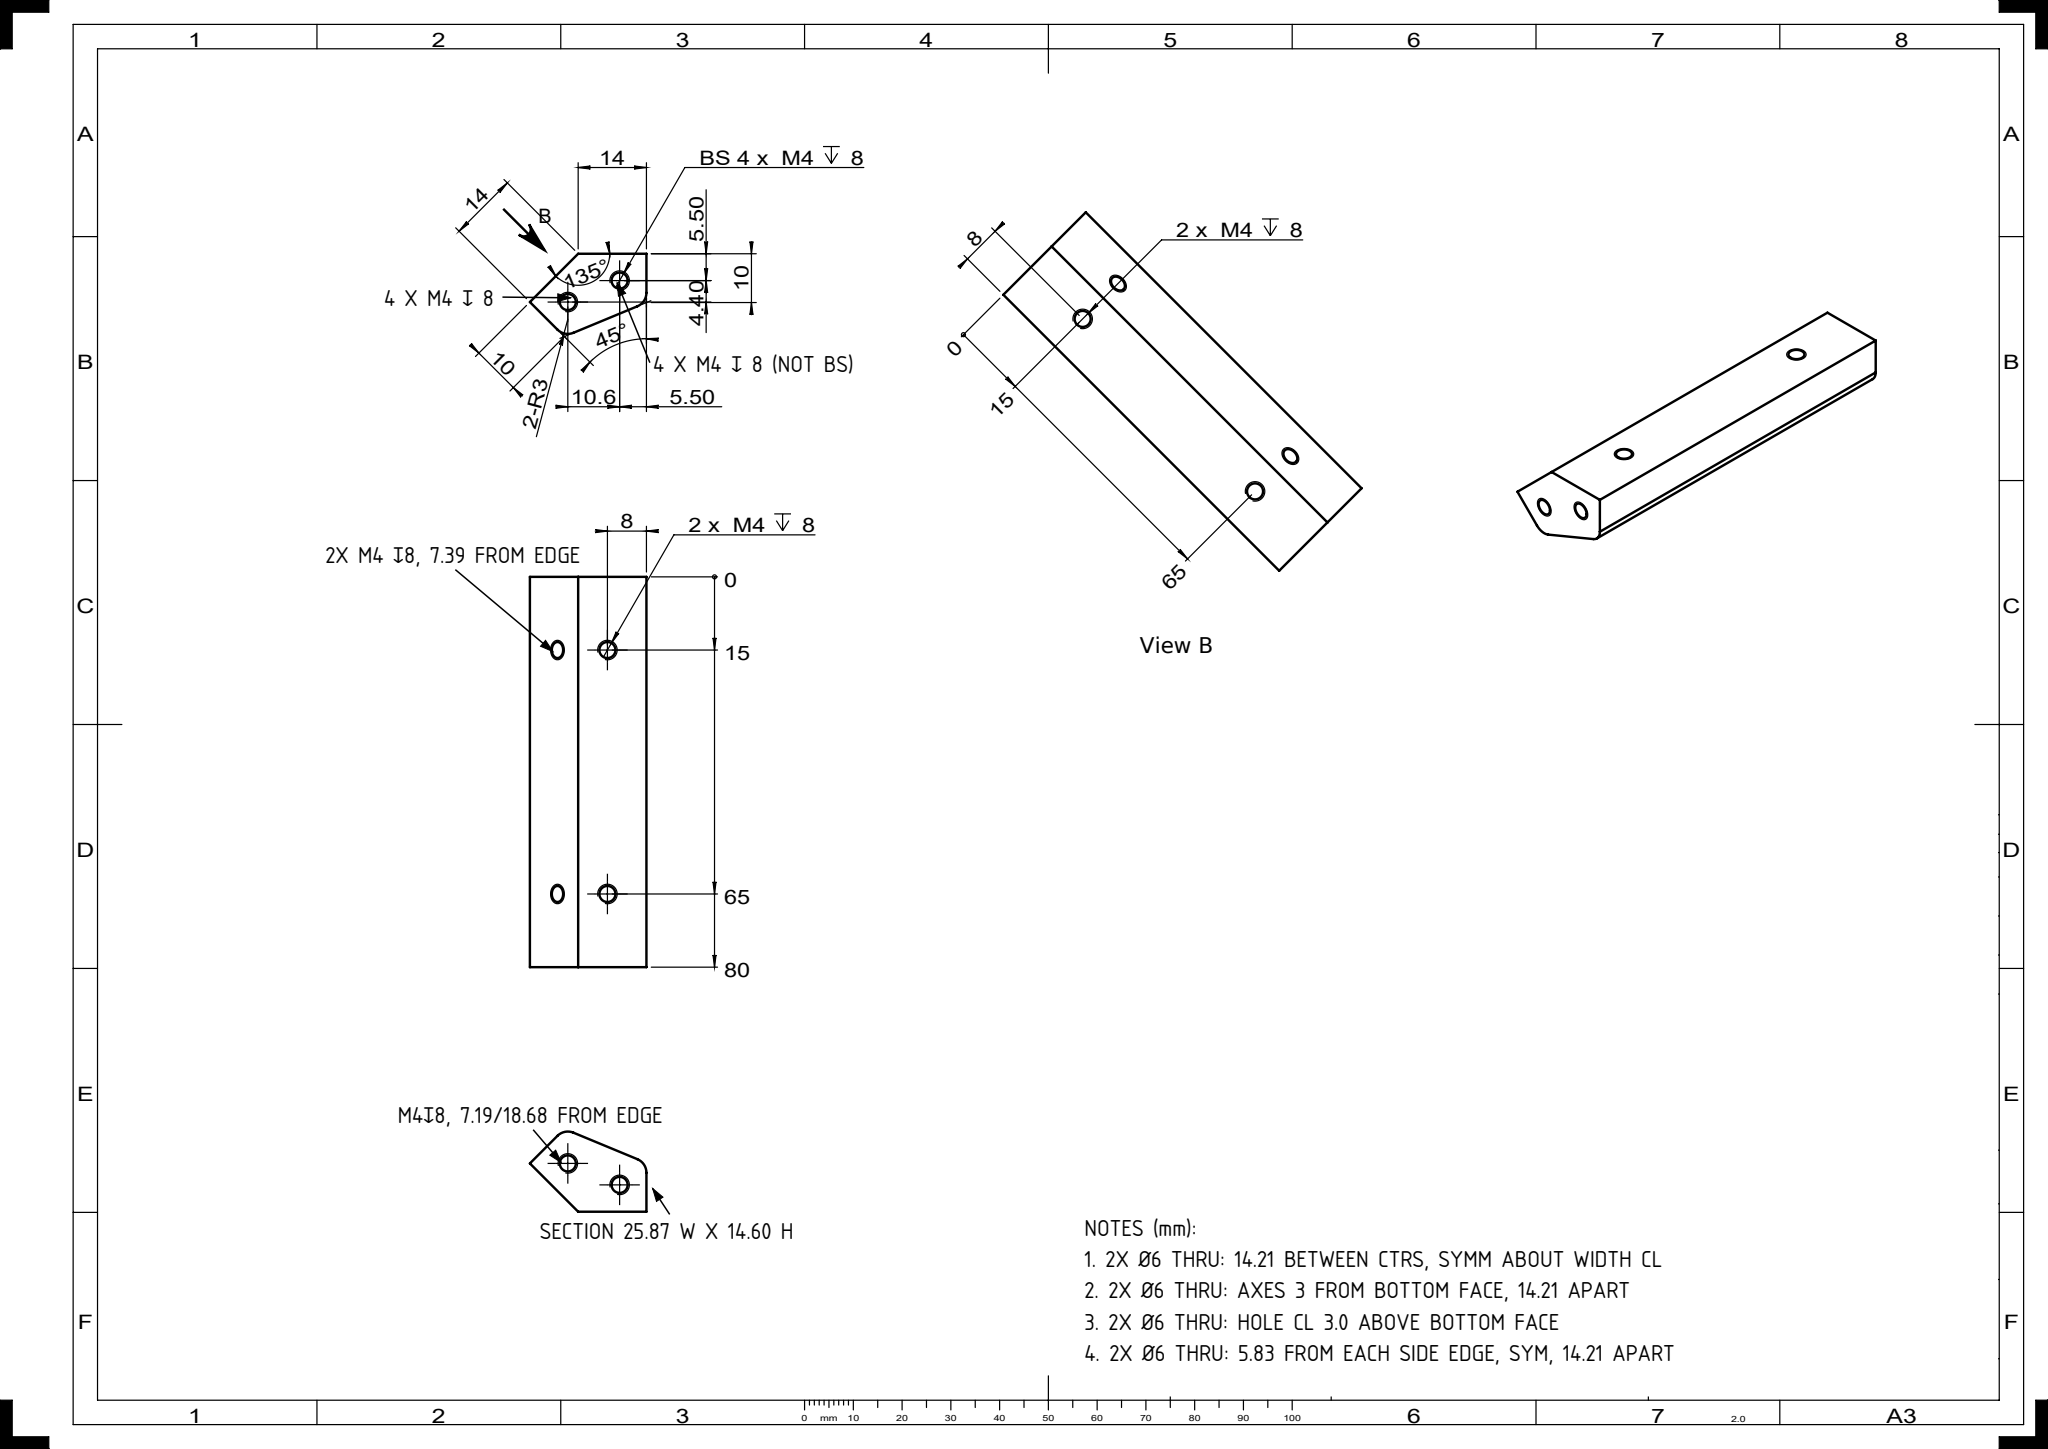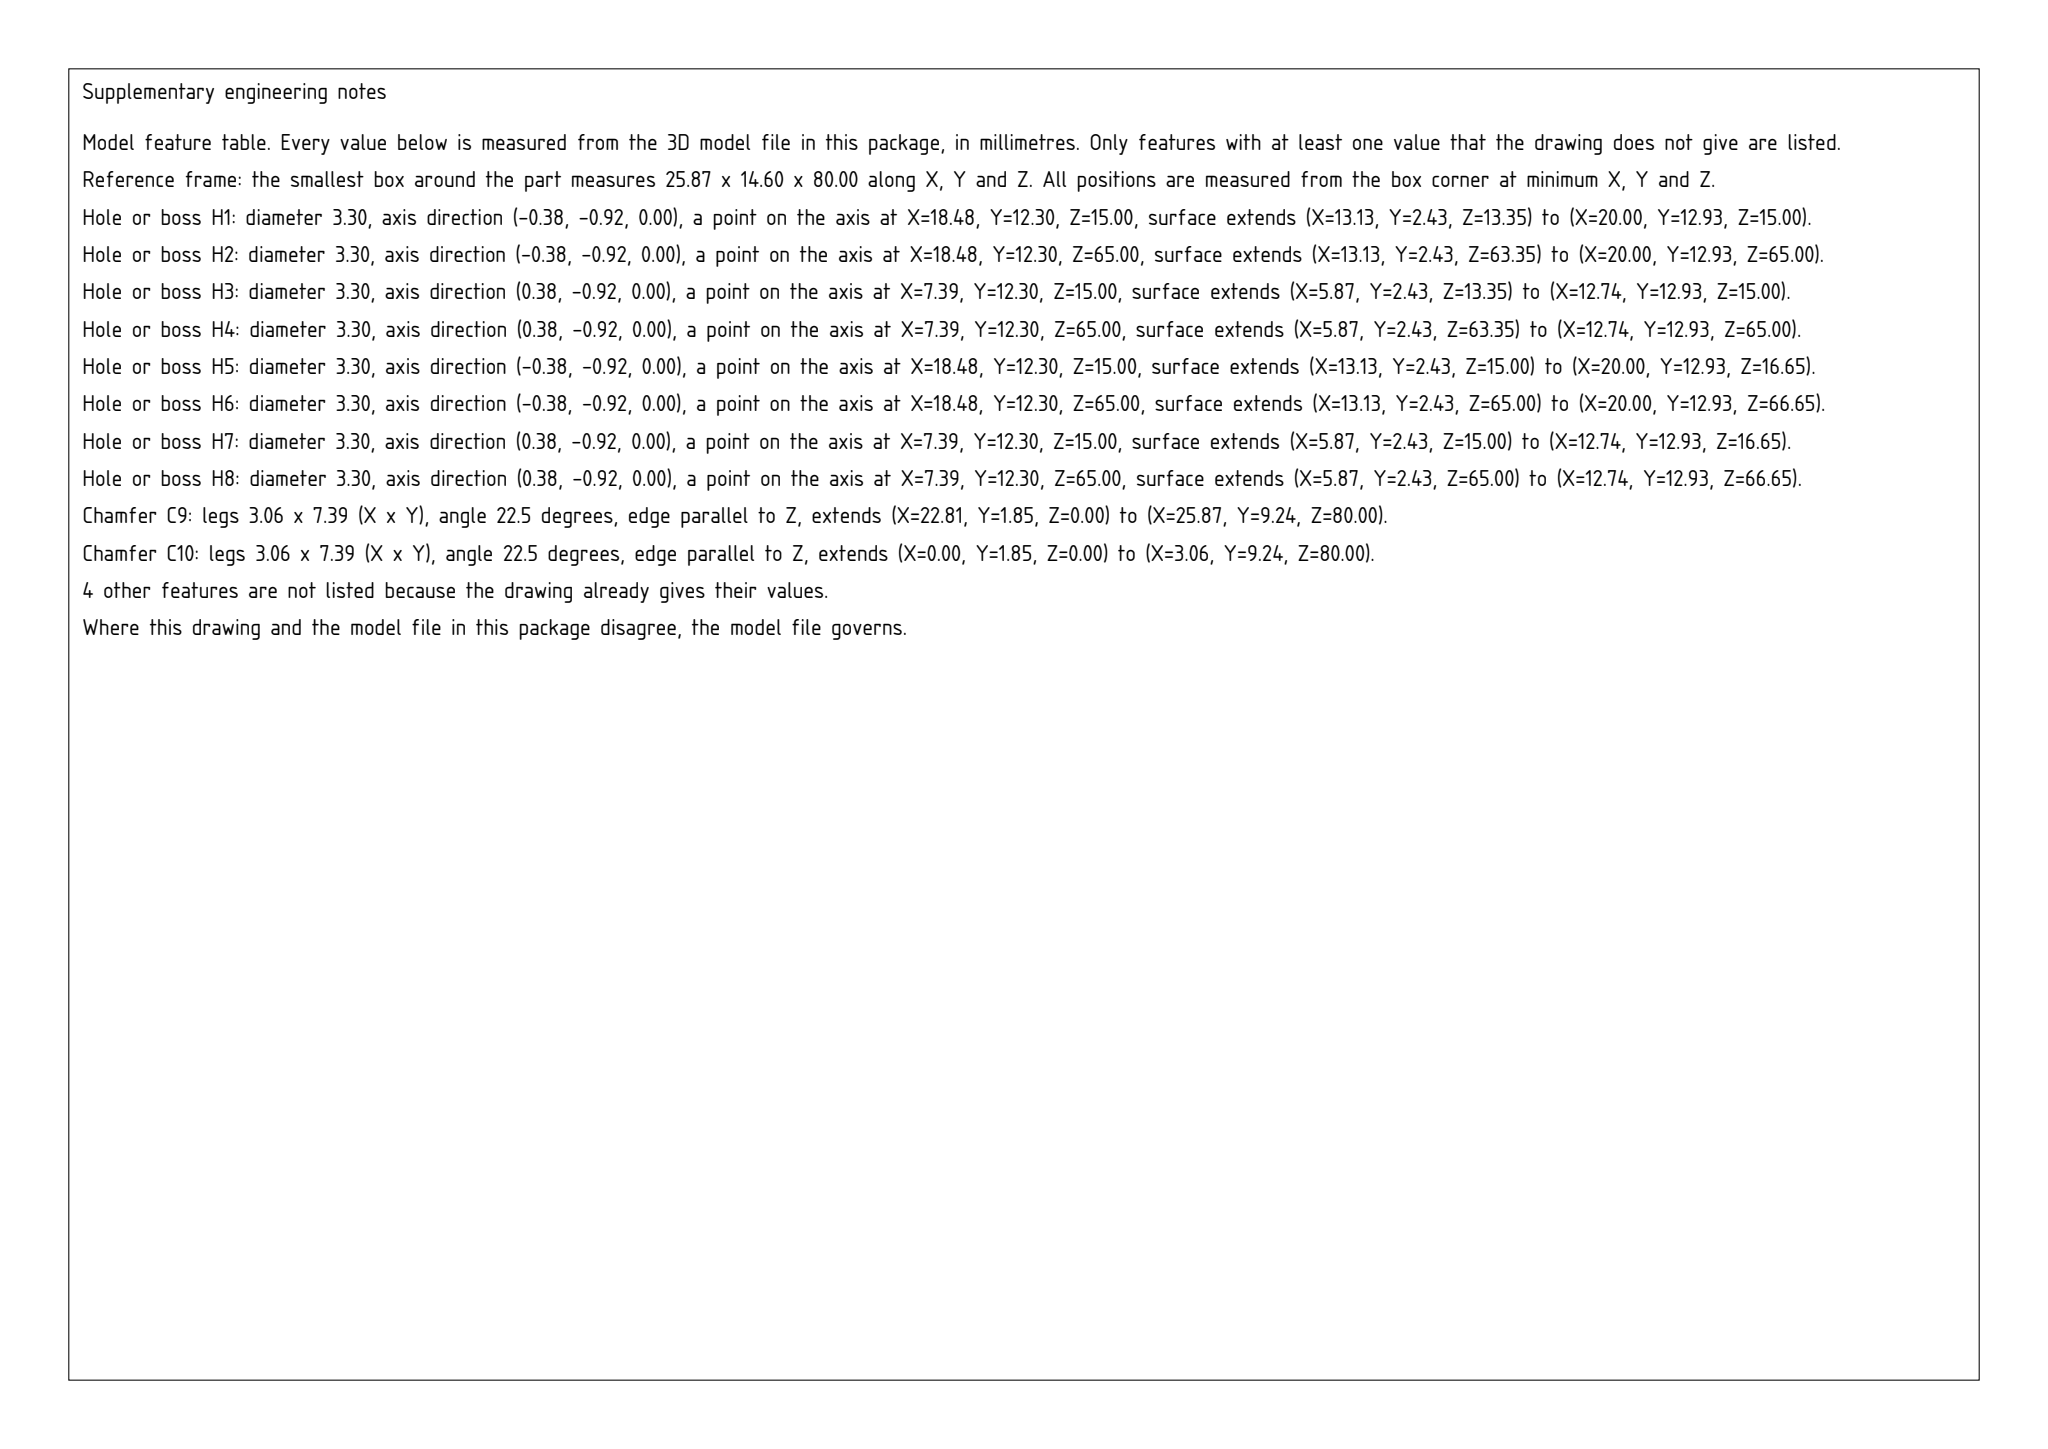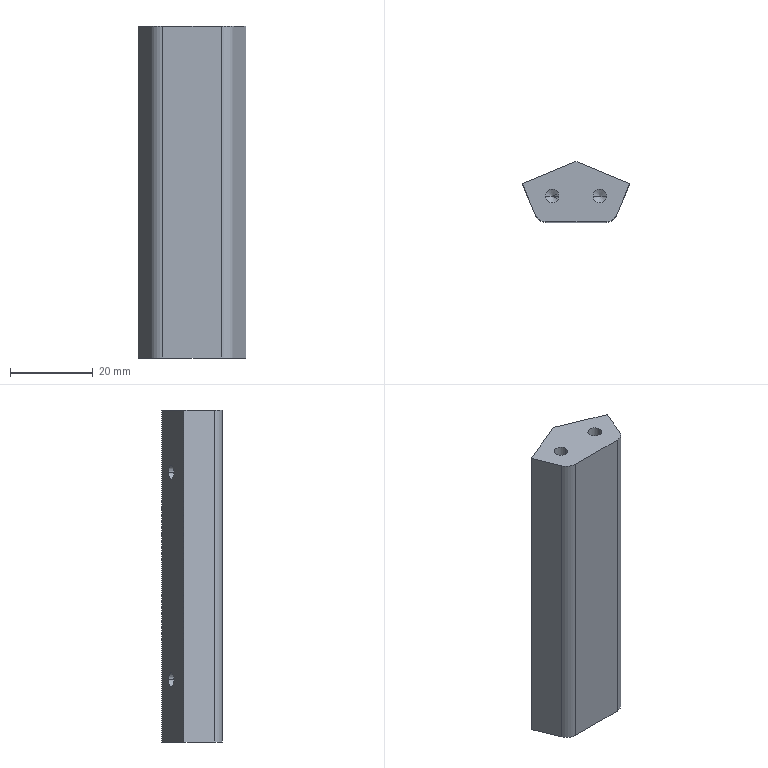Part | SolidWorks | mm | 1 solid | 41 faces | box 25.87 x 14.6 x 80 mm | volume 21014 mm3 | cylinder 18 | cone 16 | plane 7 | commonest cylinder face diameters 3.3 x16 6 x2
Drawing notes:
2X Ø6 THRU: 14.21 BETWEEN CTRS, SYMM ABOUT WIDTH CL | from the solid: Ø6 z-axis holes at x=5.83 & 20.04 (bbox x=25.869): spacing 14.21, both 5.83 from side faces
2X Ø6 THRU: AXES 3 FROM BOTTOM FACE, 14.21 APART | from the solid: Ø6 z-axis cyls at (5.83,3.0) & (20.04,3.0), L=80 THRU; y=0 plane is bottom face; spacing 20.04-5.83=14.21
DISREGARD "BS"; END HOLES READ: 4 X M4 DP 8 | from the solid: 4X Ø3.3 z-axis tapped holes at (7.19,6.26) & (18.68,6.26), drill L=10, thread depth 8
2X Ø6 THRU: HOLE CL 3.0 ABOVE BOTTOM FACE | from the solid: 6.0 dia z-axis cylinders at y=3.0 (bbox H=14.596, plane y=0)
2X Ø6 THRU: 5.83 FROM EACH SIDE EDGE, SYM, 14.21 APART | from the solid: 6.0 dia holes at x=5.83 and x=20.04; bbox W=25.869 -> 25.869-20.04=5.83
2ND ROW 2X M4 DP 8: 7.39 FROM OPP SIDE EDGE, Z=15 & 65 | from the solid: 3.3 dia y-axis holes at x=18.48, z=15 & 65; 25.869-18.48=7.39
END FACE M4 DP 8: 7.19 & 18.68 FROM SIDE EDGE, 6.26 FROM BOT | from the solid: 3.3 dia z-axis holes at (7.19,6.26) and (18.68,6.26), depth 10
SECTION OVERALL: 25.87 W X 14.60 H | from the solid: bbox_xyz 25.869 x 14.596
END VIEW THREAD NOTE READS: 4 x M4 DP 8 (DELETE 'BS') | from the solid: z-axis 3.3 dia tapped holes, 2 positions x 2 ends = 4 total, depth 10